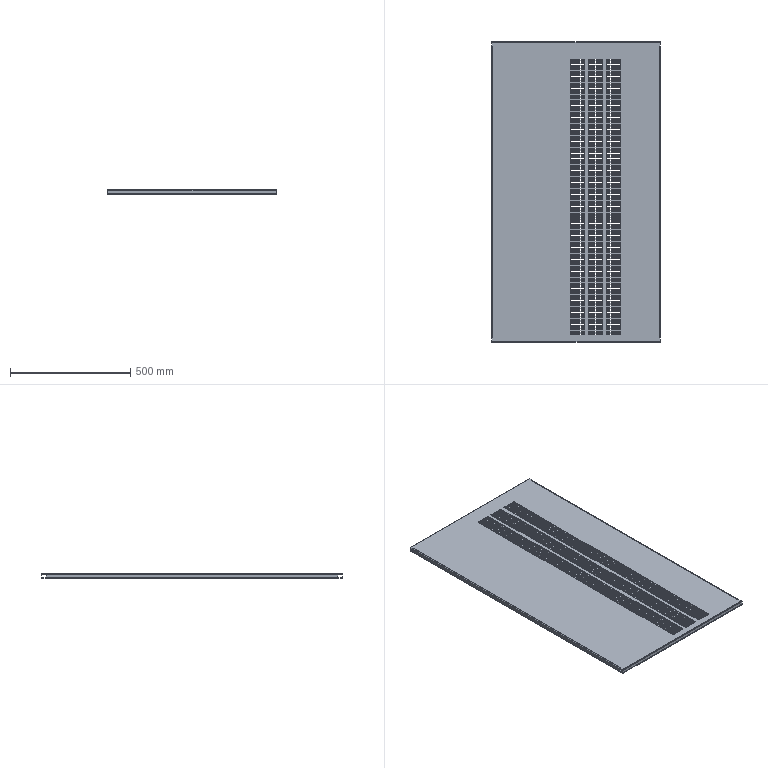Component | SolidWorks | RightEndPlate-1 | 1 solid | 1466 faces | volume 1763592 mm3 | plane 760 | cylinder 706 | commonest cylinder face diameters 5 x690 8 x8 4 x8